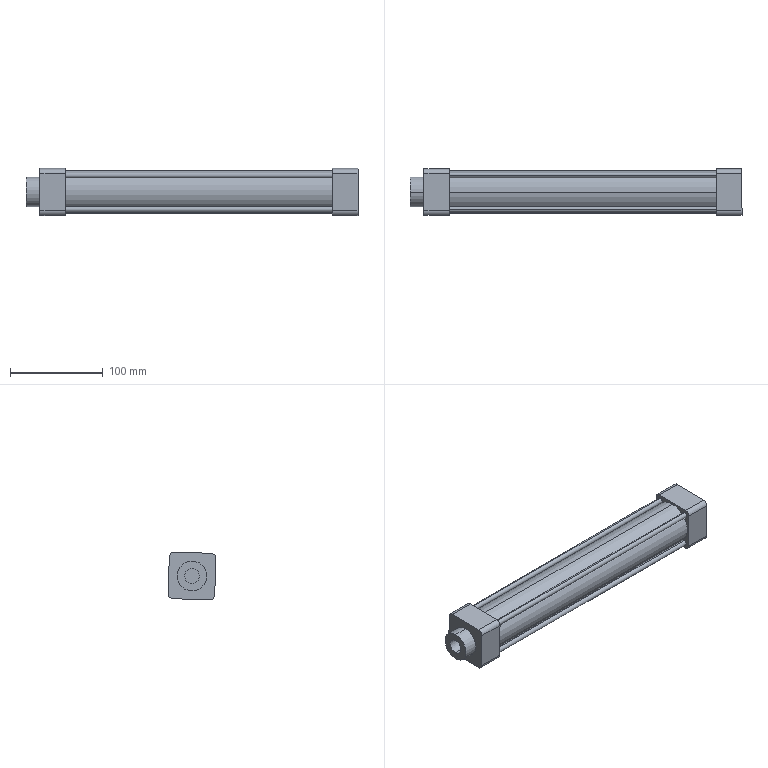Component | SolidWorks | SC40-250Cylinder-1 | 1 solid | 39 faces | volume 289127 mm3 | cylinder 24 | plane 15 | commonest cylinder face diameters 6 x8 10 x8 32 x2 46 x2 16 x2 40 x2